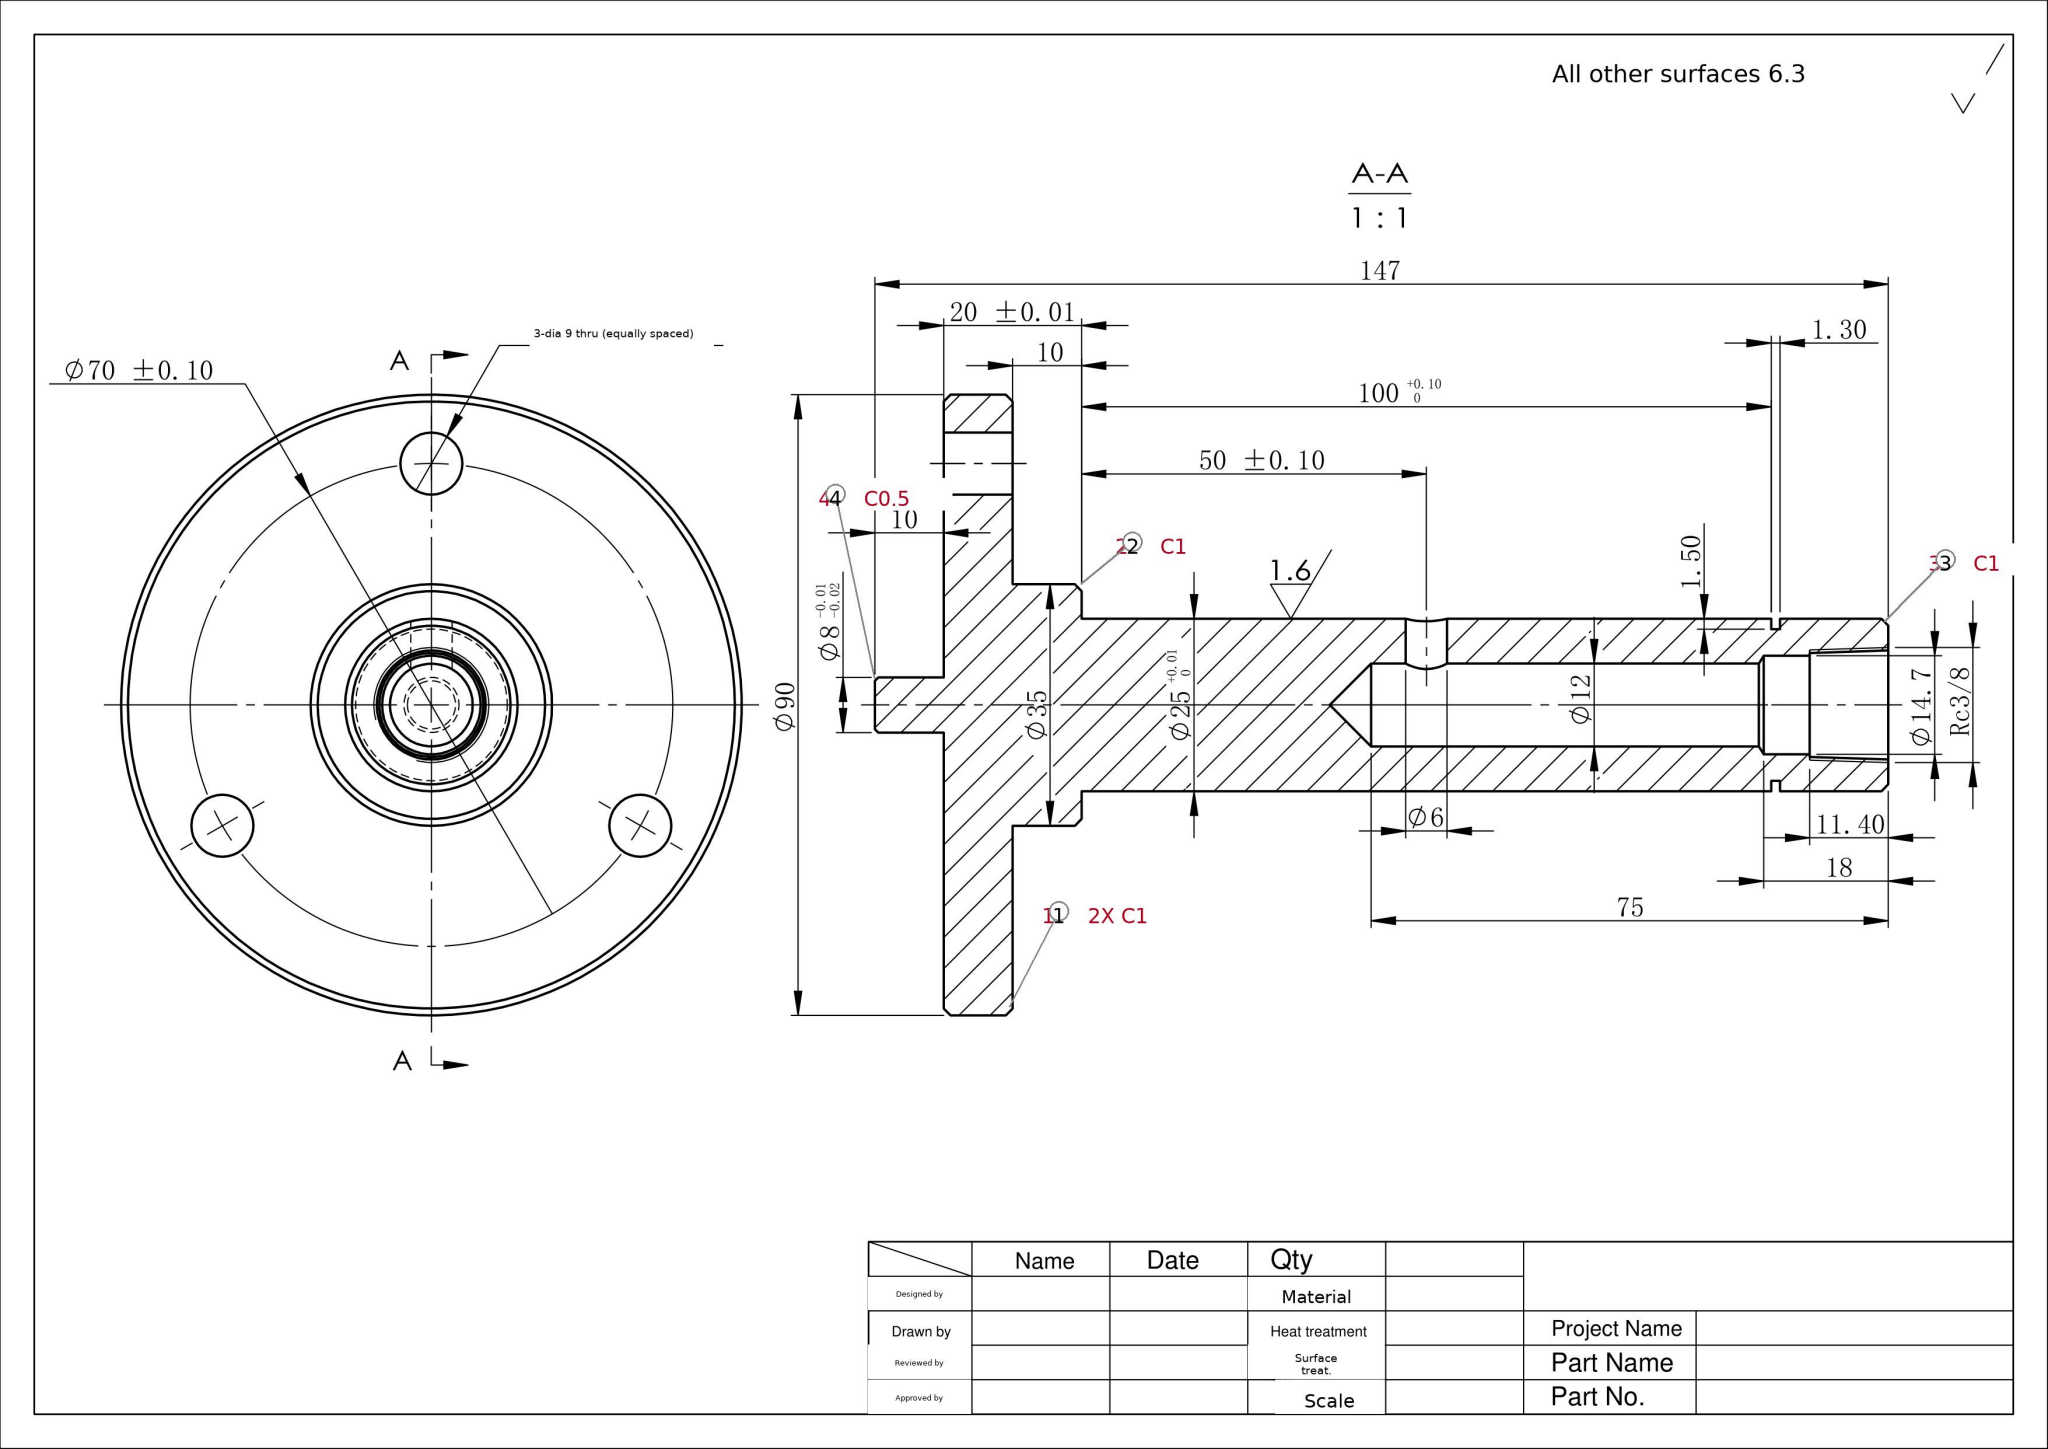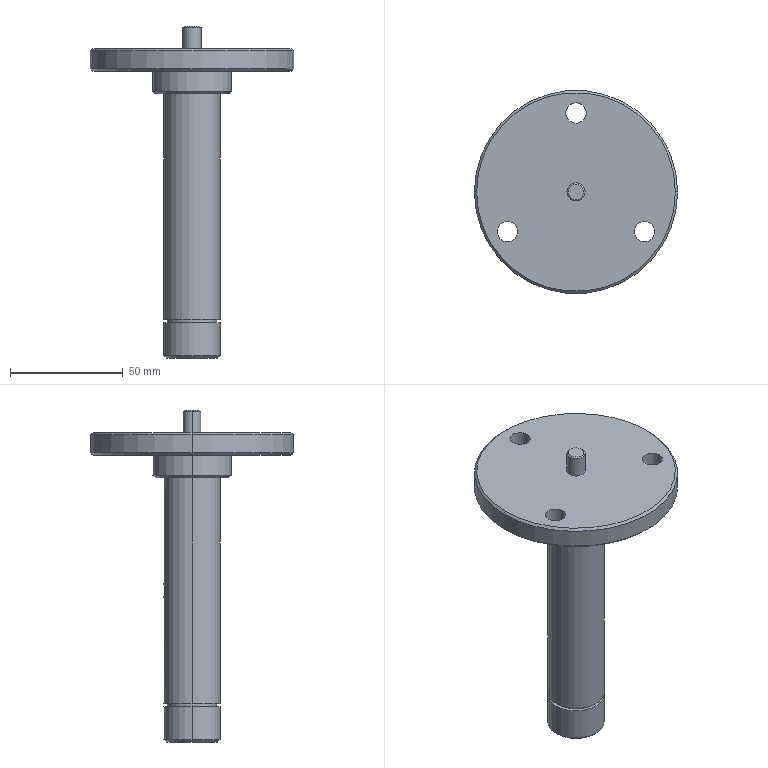Part | SolidWorks | mm | 1 solid | 48 faces | box 90 x 90 x 147 mm | volume 118668 mm3 | cylinder 24 | cone 16 | plane 8 | commonest cylinder face diameters 9 x6 25 x4 12 x2 14.3 x2 8 x2 90 x2 22 x2 6 x2
build123d program:
from build123d import *

# Parameters (mm, degrees)
SKETCH1_R          = 12.5
EXTRUDE1_DEPTH     = 127
EXTRUDE2_START     = -10
SKETCH2_R          = 17.5
SKETCH2_R_2        = 12.5
EXTRUDE2_DEPTH     = 10
SKETCH3_R          = 3
CUT_EXTRUDE1_DEPTH = 130.389
SKETCH5_W          = 9.308
SKETCH5_H          = 1.3
SKETCH6_W          = 45
SKETCH6_H          = 10
SKETCH7_R          = 4
EXTRUDE3_DEPTH     = 10
SKETCH12_R         = 6
CUT_EXTRUDE6_DEPTH = 75
SKETCH13_R         = 4.5
CUT_EXTRUDE7_DEPTH = 143.053
CIRPATTERN1_COUNT  = 3
CHAMFER1_SIZE      = 1
CHAMFER2_SIZE      = 0.5


with BuildPart() as part:
    # Sketch1 → Extrude1 (new body)
    with BuildSketch(Plane.XY):
        Circle(SKETCH1_R)
    extrude(amount=EXTRUDE1_DEPTH)

    # Sketch2 → Extrude2 (add)
    with BuildSketch(Plane.XY.offset(127).offset(EXTRUDE2_START)):
        Circle(SKETCH2_R)
        Circle(SKETCH2_R_2, mode=Mode.SUBTRACT)
    extrude(amount=EXTRUDE2_DEPTH)

    # Sketch3 → Cut-Extrude1 (cut, through all)
    with BuildSketch(Plane(origin=(0, 0, 0), x_dir=(1, 0, 0), z_dir=(0, 1, 0))):
        with Locations(Location((0, -67, 0), (0, 0, 90))):
            Circle(SKETCH3_R)
    extrude(amount=CUT_EXTRUDE1_DEPTH, mode=Mode.SUBTRACT)

    # Sketch5 → Cut-Revolve1 (revolve, cut)
    with BuildSketch(Plane(origin=(0, 0, 0), x_dir=(1, 0, 0), z_dir=(0, 1, 0)), mode=Mode.PRIVATE) as cut_revolve1_sk:
        with Locations((15.654, -16.35)):
            Rectangle(SKETCH5_W, SKETCH5_H)
    revolve(cut_revolve1_sk.sketch.rotate(Axis((0, 0, 0), (0, 0, 1)), 180), axis=Axis((0, 0, 0), (0, 0, 1)), mode=Mode.SUBTRACT)

    # Sketch6 → Revolve1 (revolve)
    with BuildSketch(Plane(origin=(0, 0, 0), x_dir=(1, 0, 0), z_dir=(0, 1, 0)), mode=Mode.PRIVATE) as revolve1_sk:
        with Locations((22.5, -132)):
            Rectangle(SKETCH6_W, SKETCH6_H)
    revolve(revolve1_sk.sketch.rotate(Axis((0, 0, 0), (0, 0, 1)), 180), axis=Axis((0, 0, 0), (0, 0, 1)))

    # Sketch7 → Extrude3 (add)
    with BuildSketch(Plane.XY.offset(137)):
        with Locations(Location((0, 0, 0), (0, 0, 180))):
            Circle(SKETCH7_R)
    extrude(amount=EXTRUDE3_DEPTH)

    # Sketch11 → 3_8 Rc Tapped Hole1 (revolve, cut)
    with BuildSketch(Plane.YZ):
        Polygon((0, 0), (0, 22.386), (7.15, 18.09), (7.15, 11.4), (7.547, 11.4), (7.903, 0), align=None)
    revolve(axis=Axis((0, 0, -6.35), (0, 0, 1)), mode=Mode.SUBTRACT)

    # Sketch12 → Cut-Extrude6 (cut)
    with BuildSketch(Plane(origin=(0, 0, 0), x_dir=(-1, 0, 0), z_dir=(0, 0, -1))):
        Circle(SKETCH12_R)
    extrude(amount=-CUT_EXTRUDE6_DEPTH, mode=Mode.SUBTRACT)

    # Sketch13 → Cut-Extrude7 (cut, through all)
    with BuildSketch(Plane(origin=(0, 0, 127), x_dir=(-1, 0, 0), z_dir=(0, 0, -1))):
        with Locations((0, 35)):
            Circle(SKETCH13_R)
    cut_extrude7 = extrude(amount=-CUT_EXTRUDE7_DEPTH, mode=Mode.SUBTRACT)

    # CirPattern1: Cut-Extrude7 ×3 about axis
    cirpattern1_axis = Axis((0, 0, 0), (0, 0, 1))
    for i in range(1, CIRPATTERN1_COUNT):
        add(cut_extrude7.rotate(cirpattern1_axis, i * 360 / CIRPATTERN1_COUNT), mode=Mode.SUBTRACT)

    # Sketch14 → Cut-Revolve2 (revolve, cut)
    with BuildSketch(Plane(origin=(0, 0, 0), x_dir=(0, 0, -1), z_dir=(1, 0, 0)), mode=Mode.PRIVATE) as cut_revolve2_sk:
        Polygon((-75, 6), (-81, 0), (-75, 0), align=None)
    revolve(cut_revolve2_sk.sketch.rotate(Axis((0, 0, 0), (0, 0, 1)), 90), axis=Axis((0, 0, 0), (0, 0, 1)), mode=Mode.SUBTRACT)

    # Chamfer1
    chamfer1_edges = [part.edges().sort_by_distance(p)[0] for p in [
        (-12.5, 0, 0),
        (45, 0, 127),
        (45, 0, 137),
        (-17.5, 0, 117),
    ]]
    chamfer(chamfer1_edges, length=CHAMFER1_SIZE)

    # Chamfer2
    chamfer2_edges = [part.edges().sort_by_distance(p)[0] for p in [
        (4, 0, 147),
    ]]
    chamfer(chamfer2_edges, length=CHAMFER2_SIZE)


solid = part.part